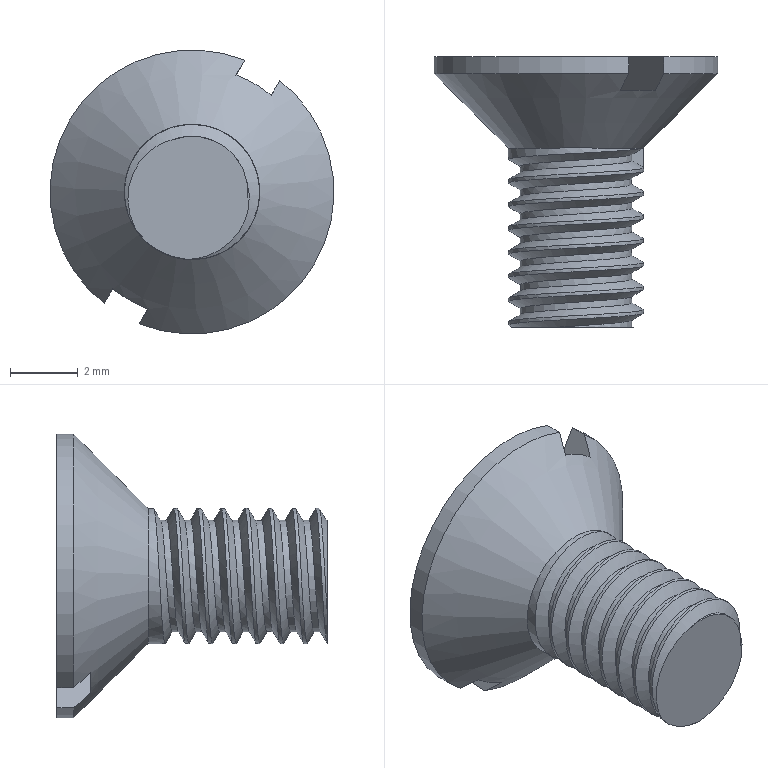Component | NX | SCREW_2 | 1 solid | 15 faces | volume 142 mm3 | plane 7 | cylinder 4 | spline 3 | cone 1 | commonest cylinder face diameters 8.4 x2 4 x1 3.3 x1